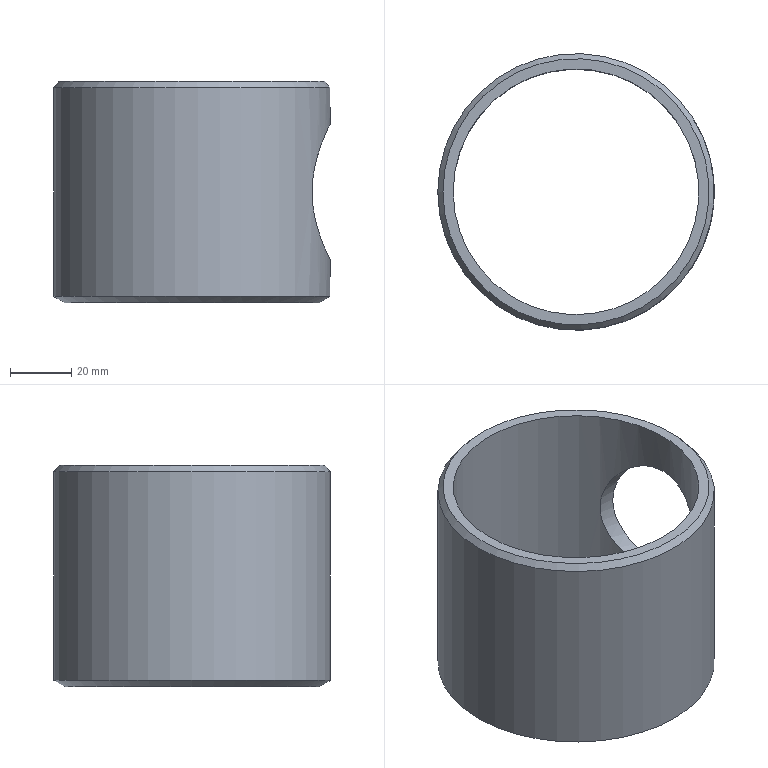Component | NX | CH3404_19_3-3 | 1 solid | 7 faces | box 90 x 90 x 72 mm | volume 86640 mm3 | cylinder 3 | cone 2 | plane 2 | commonest cylinder face diameters 90 x1 80 x1 44.5 x1
STEP:
#1=CARTESIAN_POINT('',(0.,0.,0.));
#2=DIRECTION('',(0.,0.,1.));
#3=DIRECTION('',(1.,0.,0.));
#4=AXIS2_PLACEMENT_3D('',#1,#2,#3);
#5=CARTESIAN_POINT('',(-45.,0.,74.));
#6=VERTEX_POINT('',#5);
#7=CARTESIAN_POINT('',(0.,0.,74.));
#8=DIRECTION('',(0.,0.,-1.));
#9=DIRECTION('',(-1.,0.,0.));
#10=AXIS2_PLACEMENT_3D('',#7,#8,#9);
#11=CIRCLE('',#10,45.);
#12=CARTESIAN_POINT('',(0.,0.,4.));
#13=DIRECTION('',(0.,0.,-1.));
#14=DIRECTION('',(-1.,0.,0.));
#15=AXIS2_PLACEMENT_3D('',#12,#13,#14);
#16=CYLINDRICAL_SURFACE('',#15,45.);
#17=CARTESIAN_POINT('',(0.,-70.));
#18=DIRECTION('',(1.,0.));
#19=VECTOR('',#18,1.);
#20=LINE('',#17,#19);
#21=(GEOMETRIC_REPRESENTATION_CONTEXT(2)PARAMETRIC_REPRESENTATION_CONTEXT()REPRESENTATION_CONTEXT('',''));
#22=DEFINITIONAL_REPRESENTATION('',(#20),#21);
#23=PCURVE('',#16,#22);
#24=CARTESIAN_POINT('',(0.,0.,76.));
#25=DIRECTION('',(0.,0.,-1.));
#26=DIRECTION('',(-1.,0.,0.));
#27=AXIS2_PLACEMENT_3D('',#24,#25,#26);
#28=CONICAL_SURFACE('',#27,43.322,0.6981);
#29=CARTESIAN_POINT('',(0.,2.));
#30=DIRECTION('',(1.,0.));
#31=VECTOR('',#30,1.);
#32=LINE('',#29,#31);
#33=(GEOMETRIC_REPRESENTATION_CONTEXT(2)PARAMETRIC_REPRESENTATION_CONTEXT()REPRESENTATION_CONTEXT('',''));
#34=DEFINITIONAL_REPRESENTATION('',(#32),#33);
#35=PCURVE('',#28,#34);
#36=SURFACE_CURVE('',#11,(#23,#35),.PCURVE_S1.);
#37=EDGE_CURVE('',#6,#6,#36,.T.);
#38=ORIENTED_EDGE('',*,*,#37,.T.);
#39=CARTESIAN_POINT('',(-45.,0.,6.));
#40=VERTEX_POINT('',#39);
#41=CARTESIAN_POINT('',(-45.,0.,74.));
#42=CARTESIAN_POINT('',(-45.,0.,6.));
#43=B_SPLINE_CURVE_WITH_KNOTS('',1,(#41,#42),.UNSPECIFIED.,.F.,.F.,(2,2),(-70.,-2.),.PIECEWISE_BEZIER_KNOTS.);
#44=CARTESIAN_POINT('',(6.283,0.));
#45=DIRECTION('',(0.,1.));
#46=VECTOR('',#45,1.);
#47=LINE('',#44,#46);
#48=(GEOMETRIC_REPRESENTATION_CONTEXT(2)PARAMETRIC_REPRESENTATION_CONTEXT()REPRESENTATION_CONTEXT('',''));
#49=DEFINITIONAL_REPRESENTATION('',(#47),#48);
#50=PCURVE('',#16,#49);
#51=CARTESIAN_POINT('',(0.,0.));
#52=DIRECTION('',(0.,1.));
#53=VECTOR('',#52,1.);
#54=LINE('',#51,#53);
#55=(GEOMETRIC_REPRESENTATION_CONTEXT(2)PARAMETRIC_REPRESENTATION_CONTEXT()REPRESENTATION_CONTEXT('',''));
#56=DEFINITIONAL_REPRESENTATION('',(#54),#55);
#57=PCURVE('',#16,#56);
#58=SEAM_CURVE('',#43,(#50,#57),.PCURVE_S1.);
#59=EDGE_CURVE('',#6,#40,#58,.T.);
#60=ORIENTED_EDGE('',*,*,#59,.T.);
#61=CARTESIAN_POINT('',(0.,0.,6.));
#62=DIRECTION('',(0.,0.,-1.));
#63=DIRECTION('',(-1.,0.,0.));
#64=AXIS2_PLACEMENT_3D('',#61,#62,#63);
#65=CIRCLE('',#64,45.);
#66=CARTESIAN_POINT('',(0.,-2.));
#67=DIRECTION('',(1.,0.));
#68=VECTOR('',#67,1.);
#69=LINE('',#66,#68);
#70=(GEOMETRIC_REPRESENTATION_CONTEXT(2)PARAMETRIC_REPRESENTATION_CONTEXT()REPRESENTATION_CONTEXT('',''));
#71=DEFINITIONAL_REPRESENTATION('',(#69),#70);
#72=PCURVE('',#16,#71);
#73=CARTESIAN_POINT('',(0.,0.,6.));
#74=DIRECTION('',(0.,0.,1.));
#75=DIRECTION('',(1.,0.,0.));
#76=AXIS2_PLACEMENT_3D('',#73,#74,#75);
#77=CONICAL_SURFACE('',#76,45.,1.047);
#78=CARTESIAN_POINT('',(9.425,0.));
#79=DIRECTION('',(-1.,0.));
#80=VECTOR('',#79,1.);
#81=LINE('',#78,#80);
#82=(GEOMETRIC_REPRESENTATION_CONTEXT(2)PARAMETRIC_REPRESENTATION_CONTEXT()REPRESENTATION_CONTEXT('',''));
#83=DEFINITIONAL_REPRESENTATION('',(#81),#82);
#84=PCURVE('',#77,#83);
#85=SURFACE_CURVE('',#65,(#72,#84),.PCURVE_S1.);
#86=EDGE_CURVE('',#40,#40,#85,.T.);
#87=ORIENTED_EDGE('',*,*,#86,.F.);
#88=ORIENTED_EDGE('',*,*,#59,.F.);
#89=EDGE_LOOP('',(#38,#60,#87,#88));
#90=FACE_BOUND('',#89,.T.);
#91=CARTESIAN_POINT('',(45.,0.,62.25));
#92=VERTEX_POINT('',#91);
#93=CARTESIAN_POINT('',(45.,2.991,62.25));
#94=CARTESIAN_POINT('',(45.,-2.991,62.25));
#95=CARTESIAN_POINT('',(44.693,-5.921,61.644));
#96=CARTESIAN_POINT('',(43.646,-11.292,59.392));
#97=CARTESIAN_POINT('',(42.91,-13.724,57.744));
#98=CARTESIAN_POINT('',(41.405,-17.756,53.708));
#99=CARTESIAN_POINT('',(40.626,-19.394,51.281));
#100=CARTESIAN_POINT('',(39.48,-21.631,45.957));
#101=CARTESIAN_POINT('',(39.118,-22.243,43.008));
#102=CARTESIAN_POINT('',(39.111,-22.257,37.093));
#103=CARTESIAN_POINT('',(39.464,-21.66,34.132));
#104=CARTESIAN_POINT('',(40.617,-19.412,28.742));
#105=CARTESIAN_POINT('',(41.395,-17.778,26.32));
#106=CARTESIAN_POINT('',(42.902,-13.75,22.276));
#107=CARTESIAN_POINT('',(43.64,-11.311,20.622));
#108=CARTESIAN_POINT('',(44.684,-5.978,18.374));
#109=CARTESIAN_POINT('',(44.996,-3.009,17.758));
#110=CARTESIAN_POINT('',(45.004,2.891,17.742));
#111=CARTESIAN_POINT('',(44.704,5.848,18.332));
#112=CARTESIAN_POINT('',(43.652,11.275,20.594));
#113=CARTESIAN_POINT('',(42.919,13.697,22.233));
#114=CARTESIAN_POINT('',(41.408,17.751,26.282));
#115=CARTESIAN_POINT('',(40.628,19.39,28.711));
#116=CARTESIAN_POINT('',(39.481,21.629,34.035));
#117=CARTESIAN_POINT('',(39.118,22.243,37.003));
#118=CARTESIAN_POINT('',(39.111,22.257,42.892));
#119=CARTESIAN_POINT('',(39.464,21.661,45.861));
#120=CARTESIAN_POINT('',(40.614,19.418,51.247));
#121=CARTESIAN_POINT('',(41.392,17.788,53.672));
#122=CARTESIAN_POINT('',(42.911,13.725,57.747));
#123=CARTESIAN_POINT('',(43.643,11.303,59.385));
#124=CARTESIAN_POINT('',(44.69,5.936,61.64));
#125=CARTESIAN_POINT('',(45.,2.991,62.25));
#126=CARTESIAN_POINT('',(45.,-2.991,62.25));
#127=B_SPLINE_CURVE_WITH_KNOTS('',3,(#93,#94,#95,#96,#97,#98,#99,#100,#101,#102,#103,#104,#105,#106,#107,#108,#109,#110,#111,#112,#113,#114,#115,#116,#117,#118,#119,#120,#121,#122,#123,#124,#125,#126),.UNSPECIFIED.,.T.,.F.,(2,2,2,2,2,2,2,2,2,2,2,2,2,2,2,2,2,2,2),(-0.0625,0.,0.0625,0.125,0.1875,0.25,0.3125,0.375,0.4375,0.5,0.5625,0.625,0.6875,0.75,0.8125,0.875,0.9375,1.,1.062),.UNSPECIFIED.);
#128=CARTESIAN_POINT('',(3.142,-58.25));
#129=CARTESIAN_POINT('',(3.158,-58.25));
#130=CARTESIAN_POINT('',(3.19,-58.179));
#131=CARTESIAN_POINT('',(3.237,-57.866));
#132=CARTESIAN_POINT('',(3.284,-57.354));
#133=CARTESIAN_POINT('',(3.329,-56.65));
#134=CARTESIAN_POINT('',(3.372,-55.761));
#135=CARTESIAN_POINT('',(3.414,-54.7));
#136=CARTESIAN_POINT('',(3.454,-53.479));
#137=CARTESIAN_POINT('',(3.491,-52.111));
#138=CARTESIAN_POINT('',(3.525,-50.608));
#139=CARTESIAN_POINT('',(3.556,-48.97));
#140=CARTESIAN_POINT('',(3.584,-47.214));
#141=CARTESIAN_POINT('',(3.608,-45.354));
#142=CARTESIAN_POINT('',(3.627,-43.405));
#143=CARTESIAN_POINT('',(3.643,-41.367));
#144=CARTESIAN_POINT('',(3.653,-39.266));
#145=CARTESIAN_POINT('',(3.659,-37.127));
#146=CARTESIAN_POINT('',(3.659,-34.974));
#147=CARTESIAN_POINT('',(3.654,-32.83));
#148=CARTESIAN_POINT('',(3.643,-30.72));
#149=CARTESIAN_POINT('',(3.628,-28.666));
#150=CARTESIAN_POINT('',(3.608,-26.692));
#151=CARTESIAN_POINT('',(3.584,-24.819));
#152=CARTESIAN_POINT('',(3.556,-23.057));
#153=CARTESIAN_POINT('',(3.525,-21.417));
#154=CARTESIAN_POINT('',(3.491,-19.912));
#155=CARTESIAN_POINT('',(3.454,-18.541));
#156=CARTESIAN_POINT('',(3.415,-17.317));
#157=CARTESIAN_POINT('',(3.373,-16.254));
#158=CARTESIAN_POINT('',(3.33,-15.367));
#159=CARTESIAN_POINT('',(3.285,-14.662));
#160=CARTESIAN_POINT('',(3.238,-14.146));
#161=CARTESIAN_POINT('',(3.191,-13.827));
#162=CARTESIAN_POINT('',(3.143,-13.715));
#163=CARTESIAN_POINT('',(3.095,-13.815));
#164=CARTESIAN_POINT('',(3.048,-14.12));
#165=CARTESIAN_POINT('',(3.001,-14.627));
#166=CARTESIAN_POINT('',(2.955,-15.331));
#167=CARTESIAN_POINT('',(2.911,-16.222));
#168=CARTESIAN_POINT('',(2.87,-17.282));
#169=CARTESIAN_POINT('',(2.83,-18.502));
#170=CARTESIAN_POINT('',(2.793,-19.871));
#171=CARTESIAN_POINT('',(2.759,-21.379));
#172=CARTESIAN_POINT('',(2.727,-23.02));
#173=CARTESIAN_POINT('',(2.7,-24.778));
#174=CARTESIAN_POINT('',(2.676,-26.638));
#175=CARTESIAN_POINT('',(2.656,-28.587));
#176=CARTESIAN_POINT('',(2.64,-30.631));
#177=CARTESIAN_POINT('',(2.63,-32.736));
#178=CARTESIAN_POINT('',(2.624,-34.876));
#179=CARTESIAN_POINT('',(2.624,-37.02));
#180=CARTESIAN_POINT('',(2.629,-39.16));
#181=CARTESIAN_POINT('',(2.64,-41.271));
#182=CARTESIAN_POINT('',(2.655,-43.326));
#183=CARTESIAN_POINT('',(2.675,-45.299));
#184=CARTESIAN_POINT('',(2.699,-47.171));
#185=CARTESIAN_POINT('',(2.727,-48.936));
#186=CARTESIAN_POINT('',(2.758,-50.581));
#187=CARTESIAN_POINT('',(2.792,-52.099));
#188=CARTESIAN_POINT('',(2.829,-53.474));
#189=CARTESIAN_POINT('',(2.869,-54.696));
#190=CARTESIAN_POINT('',(2.911,-55.756));
#191=CARTESIAN_POINT('',(2.954,-56.644));
#192=CARTESIAN_POINT('',(2.999,-57.35));
#193=CARTESIAN_POINT('',(3.046,-57.864));
#194=CARTESIAN_POINT('',(3.093,-58.178));
#195=CARTESIAN_POINT('',(3.125,-58.25));
#196=CARTESIAN_POINT('',(3.142,-58.25));
#197=B_SPLINE_CURVE_WITH_KNOTS('',3,(#128,#129,#130,#131,#132,#133,#134,#135,#136,#137,#138,#139,#140,#141,#142,#143,#144,#145,#146,#147,#148,#149,#150,#151,#152,#153,#154,#155,#156,#157,#158,#159,#160,#161,#162,#163,#164,#165,#166,#167,#168,#169,#170,#171,#172,#173,#174,#175,#176,#177,#178,#179,#180,#181,#182,#183,#184,#185,#186,#187,#188,#189,#190,#191,#192,#193,#194,#195,#196),.UNSPECIFIED.,.T.,.F.,(4,1,1,1,1,1,1,1,1,1,1,1,1,1,1,1,1,1,1,1,1,1,1,1,1,1,1,1,1,1,1,1,1,1,1,1,1,1,1,1,1,1,1,1,1,1,1,1,1,1,1,1,1,1,1,1,1,1,1,1,1,1,1,1,1,1,4),(0.,0.01515,0.0303,0.04545,0.06061,0.07576,0.09091,0.1061,0.1212,0.1364,0.1515,0.1667,0.1818,0.197,0.2121,0.2273,0.2424,0.2576,0.2727,0.2879,0.303,0.3182,0.3333,0.3485,0.3636,0.3788,0.3939,0.4091,0.4242,0.4394,0.4545,0.4697,0.4848,0.5,0.5152,0.5303,0.5455,0.5606,0.5758,0.5909,0.6061,0.6212,0.6364,0.6515,0.6667,0.6818,0.697,0.7121,0.7273,0.7424,0.7576,0.7727,0.7879,0.803,0.8182,0.8333,0.8485,0.8636,0.8788,0.8939,0.9091,0.9242,0.9394,0.9545,0.9697,0.9848,1.),.QUASI_UNIFORM_KNOTS.);
#198=(GEOMETRIC_REPRESENTATION_CONTEXT(2)PARAMETRIC_REPRESENTATION_CONTEXT()REPRESENTATION_CONTEXT('',''));
#199=DEFINITIONAL_REPRESENTATION('',(#197),#198);
#200=PCURVE('',#16,#199);
#201=CARTESIAN_POINT('',(49.5,0.,40.));
#202=DIRECTION('',(-1.,0.,0.));
#203=DIRECTION('',(0.,0.,1.));
#204=AXIS2_PLACEMENT_3D('',#201,#202,#203);
#205=CYLINDRICAL_SURFACE('',#204,22.25);
#206=CARTESIAN_POINT('',(6.283,4.5));
#207=CARTESIAN_POINT('',(6.251,4.5));
#208=CARTESIAN_POINT('',(6.186,4.536));
#209=CARTESIAN_POINT('',(6.089,4.691));
#210=CARTESIAN_POINT('',(5.993,4.938));
#211=CARTESIAN_POINT('',(5.898,5.271));
#212=CARTESIAN_POINT('',(5.803,5.68));
#213=CARTESIAN_POINT('',(5.708,6.15));
#214=CARTESIAN_POINT('',(5.614,6.664));
#215=CARTESIAN_POINT('',(5.521,7.204));
#216=CARTESIAN_POINT('',(5.427,7.755));
#217=CARTESIAN_POINT('',(5.334,8.301));
#218=CARTESIAN_POINT('',(5.24,8.822));
#219=CARTESIAN_POINT('',(5.146,9.297));
#220=CARTESIAN_POINT('',(5.051,9.706));
#221=CARTESIAN_POINT('',(4.956,10.033));
#222=CARTESIAN_POINT('',(4.86,10.264));
#223=CARTESIAN_POINT('',(4.763,10.389));
#224=CARTESIAN_POINT('',(4.666,10.392));
#225=CARTESIAN_POINT('',(4.57,10.272));
#226=CARTESIAN_POINT('',(4.473,10.045));
#227=CARTESIAN_POINT('',(4.377,9.72));
#228=CARTESIAN_POINT('',(4.281,9.308));
#229=CARTESIAN_POINT('',(4.187,8.831));
#230=CARTESIAN_POINT('',(4.093,8.311));
#231=CARTESIAN_POINT('',(3.999,7.764));
#232=CARTESIAN_POINT('',(3.906,7.213));
#233=CARTESIAN_POINT('',(3.812,6.672));
#234=CARTESIAN_POINT('',(3.718,6.158));
#235=CARTESIAN_POINT('',(3.623,5.687));
#236=CARTESIAN_POINT('',(3.529,5.279));
#237=CARTESIAN_POINT('',(3.434,4.946));
#238=CARTESIAN_POINT('',(3.337,4.697));
#239=CARTESIAN_POINT('',(3.241,4.539));
#240=CARTESIAN_POINT('',(3.144,4.482));
#241=CARTESIAN_POINT('',(3.048,4.533));
#242=CARTESIAN_POINT('',(2.951,4.684));
#243=CARTESIAN_POINT('',(2.855,4.929));
#244=CARTESIAN_POINT('',(2.759,5.262));
#245=CARTESIAN_POINT('',(2.663,5.673));
#246=CARTESIAN_POINT('',(2.568,6.143));
#247=CARTESIAN_POINT('',(2.474,6.656));
#248=CARTESIAN_POINT('',(2.38,7.197));
#249=CARTESIAN_POINT('',(2.287,7.751));
#250=CARTESIAN_POINT('',(2.193,8.298));
#251=CARTESIAN_POINT('',(2.099,8.819));
#252=CARTESIAN_POINT('',(2.004,9.295));
#253=CARTESIAN_POINT('',(1.91,9.705));
#254=CARTESIAN_POINT('',(1.814,10.032));
#255=CARTESIAN_POINT('',(1.718,10.264));
#256=CARTESIAN_POINT('',(1.621,10.389));
#257=CARTESIAN_POINT('',(1.525,10.392));
#258=CARTESIAN_POINT('',(1.428,10.273));
#259=CARTESIAN_POINT('',(1.332,10.045));
#260=CARTESIAN_POINT('',(1.236,9.721));
#261=CARTESIAN_POINT('',(1.14,9.31));
#262=CARTESIAN_POINT('',(1.046,8.834));
#263=CARTESIAN_POINT('',(0.9514,8.313));
#264=CARTESIAN_POINT('',(0.8574,7.765));
#265=CARTESIAN_POINT('',(0.7634,7.209));
#266=CARTESIAN_POINT('',(0.6694,6.666));
#267=CARTESIAN_POINT('',(0.5753,6.152));
#268=CARTESIAN_POINT('',(0.4809,5.683));
#269=CARTESIAN_POINT('',(0.386,5.273));
#270=CARTESIAN_POINT('',(0.2905,4.94));
#271=CARTESIAN_POINT('',(0.1943,4.692));
#272=CARTESIAN_POINT('',(0.09753,4.536));
#273=CARTESIAN_POINT('',(0.03258,4.5));
#274=CARTESIAN_POINT('',(0.,4.5));
#275=B_SPLINE_CURVE_WITH_KNOTS('',3,(#206,#207,#208,#209,#210,#211,#212,#213,#214,#215,#216,#217,#218,#219,#220,#221,#222,#223,#224,#225,#226,#227,#228,#229,#230,#231,#232,#233,#234,#235,#236,#237,#238,#239,#240,#241,#242,#243,#244,#245,#246,#247,#248,#249,#250,#251,#252,#253,#254,#255,#256,#257,#258,#259,#260,#261,#262,#263,#264,#265,#266,#267,#268,#269,#270,#271,#272,#273,#274),.UNSPECIFIED.,.F.,.F.,(4,1,1,1,1,1,1,1,1,1,1,1,1,1,1,1,1,1,1,1,1,1,1,1,1,1,1,1,1,1,1,1,1,1,1,1,1,1,1,1,1,1,1,1,1,1,1,1,1,1,1,1,1,1,1,1,1,1,1,1,1,1,1,1,1,1,4),(0.,0.01515,0.0303,0.04545,0.06061,0.07576,0.09091,0.1061,0.1212,0.1364,0.1515,0.1667,0.1818,0.197,0.2121,0.2273,0.2424,0.2576,0.2727,0.2879,0.303,0.3182,0.3333,0.3485,0.3636,0.3788,0.3939,0.4091,0.4242,0.4394,0.4545,0.4697,0.4848,0.5,0.5152,0.5303,0.5455,0.5606,0.5758,0.5909,0.6061,0.6212,0.6364,0.6515,0.6667,0.6818,0.697,0.7121,0.7273,0.7424,0.7576,0.7727,0.7879,0.803,0.8182,0.8333,0.8485,0.8636,0.8788,0.8939,0.9091,0.9242,0.9394,0.9545,0.9697,0.9848,1.),.QUASI_UNIFORM_KNOTS.);
#276=(GEOMETRIC_REPRESENTATION_CONTEXT(2)PARAMETRIC_REPRESENTATION_CONTEXT()REPRESENTATION_CONTEXT('',''));
#277=DEFINITIONAL_REPRESENTATION('',(#275),#276);
#278=PCURVE('',#205,#277);
#279=SURFACE_CURVE('',#127,(#200,#278),.PCURVE_S1.);
#280=EDGE_CURVE('',#92,#92,#279,.T.);
#281=ORIENTED_EDGE('',*,*,#280,.F.);
#282=EDGE_LOOP('',(#281));
#283=FACE_BOUND('',#282,.T.);
#284=ADVANCED_FACE('',(#90,#283),#16,.T.);
#285=CARTESIAN_POINT('',(-40.,0.,4.));
#286=VERTEX_POINT('',#285);
#287=CARTESIAN_POINT('',(0.,0.,4.));
#288=DIRECTION('',(0.,0.,-1.));
#289=DIRECTION('',(-1.,0.,0.));
#290=AXIS2_PLACEMENT_3D('',#287,#288,#289);
#291=CIRCLE('',#290,40.);
#292=CARTESIAN_POINT('',(0.,0.,4.));
#293=DIRECTION('',(0.,0.,-1.));
#294=DIRECTION('',(-1.,0.,0.));
#295=AXIS2_PLACEMENT_3D('',#292,#293,#294);
#296=CYLINDRICAL_SURFACE('',#295,40.);
#297=CARTESIAN_POINT('',(0.,0.));
#298=DIRECTION('',(1.,0.));
#299=VECTOR('',#298,1.);
#300=LINE('',#297,#299);
#301=(GEOMETRIC_REPRESENTATION_CONTEXT(2)PARAMETRIC_REPRESENTATION_CONTEXT()REPRESENTATION_CONTEXT('',''));
#302=DEFINITIONAL_REPRESENTATION('',(#300),#301);
#303=PCURVE('',#296,#302);
#304=CARTESIAN_POINT('',(0.,-41.536,4.));
#305=DIRECTION('',(0.,0.,1.));
#306=DIRECTION('',(1.,0.,0.));
#307=AXIS2_PLACEMENT_3D('',#304,#305,#306);
#308=PLANE('',#307);
#309=CARTESIAN_POINT('',(-40.,41.536));
#310=CARTESIAN_POINT('',(-40.,110.818));
#311=CARTESIAN_POINT('',(20.,76.177));
#312=CARTESIAN_POINT('',(80.,41.536));
#313=CARTESIAN_POINT('',(20.,6.895));
#314=CARTESIAN_POINT('',(-40.,-27.746));
#315=CARTESIAN_POINT('',(-40.,41.536));
#316=(BOUNDED_CURVE()B_SPLINE_CURVE(2,(#309,#310,#311,#312,#313,#314,#315),.UNSPECIFIED.,.T.,.F.)B_SPLINE_CURVE_WITH_KNOTS((1,2,2,2,2,1),(-2.094,0.,2.094,4.189,6.283,8.378),.UNSPECIFIED.)CURVE()GEOMETRIC_REPRESENTATION_ITEM()RATIONAL_B_SPLINE_CURVE((1.,0.5,1.,0.5,1.,0.5,1.))REPRESENTATION_ITEM(''));
#317=(GEOMETRIC_REPRESENTATION_CONTEXT(2)PARAMETRIC_REPRESENTATION_CONTEXT()REPRESENTATION_CONTEXT('',''));
#318=DEFINITIONAL_REPRESENTATION('',(#316),#317);
#319=PCURVE('',#308,#318);
#320=SURFACE_CURVE('',#291,(#303,#319),.PCURVE_S1.);
#321=EDGE_CURVE('',#286,#286,#320,.T.);
#322=ORIENTED_EDGE('',*,*,#321,.F.);
#323=CARTESIAN_POINT('',(-40.,0.,76.));
#324=VERTEX_POINT('',#323);
#325=CARTESIAN_POINT('',(-40.,-0.,76.));
#326=CARTESIAN_POINT('',(-40.,-0.,4.));
#327=B_SPLINE_CURVE_WITH_KNOTS('',1,(#325,#326),.UNSPECIFIED.,.F.,.F.,(2,2),(-72.,0.),.PIECEWISE_BEZIER_KNOTS.);
#328=CARTESIAN_POINT('',(0.,0.));
#329=DIRECTION('',(0.,1.));
#330=VECTOR('',#329,1.);
#331=LINE('',#328,#330);
#332=(GEOMETRIC_REPRESENTATION_CONTEXT(2)PARAMETRIC_REPRESENTATION_CONTEXT()REPRESENTATION_CONTEXT('',''));
#333=DEFINITIONAL_REPRESENTATION('',(#331),#332);
#334=PCURVE('',#296,#333);
#335=CARTESIAN_POINT('',(6.283,0.));
#336=DIRECTION('',(0.,1.));
#337=VECTOR('',#336,1.);
#338=LINE('',#335,#337);
#339=(GEOMETRIC_REPRESENTATION_CONTEXT(2)PARAMETRIC_REPRESENTATION_CONTEXT()REPRESENTATION_CONTEXT('',''));
#340=DEFINITIONAL_REPRESENTATION('',(#338),#339);
#341=PCURVE('',#296,#340);
#342=SEAM_CURVE('',#327,(#334,#341),.PCURVE_S1.);
#343=EDGE_CURVE('',#324,#286,#342,.T.);
#344=ORIENTED_EDGE('',*,*,#343,.F.);
#345=CARTESIAN_POINT('',(0.,0.,76.));
#346=DIRECTION('',(0.,0.,-1.));
#347=DIRECTION('',(-1.,0.,0.));
#348=AXIS2_PLACEMENT_3D('',#345,#346,#347);
#349=CIRCLE('',#348,40.);
#350=CARTESIAN_POINT('',(0.,-72.));
#351=DIRECTION('',(1.,0.));
#352=VECTOR('',#351,1.);
#353=LINE('',#350,#352);
#354=(GEOMETRIC_REPRESENTATION_CONTEXT(2)PARAMETRIC_REPRESENTATION_CONTEXT()REPRESENTATION_CONTEXT('',''));
#355=DEFINITIONAL_REPRESENTATION('',(#353),#354);
#356=PCURVE('',#296,#355);
#357=CARTESIAN_POINT('',(0.,-40.,76.));
#358=DIRECTION('',(0.,0.,-1.));
#359=DIRECTION('',(-1.,0.,0.));
#360=AXIS2_PLACEMENT_3D('',#357,#358,#359);
#361=PLANE('',#360);
#362=CARTESIAN_POINT('',(0.,40.));
#363=DIRECTION('',(1.,0.));
#364=AXIS2_PLACEMENT_2D('',#362,#363);
#365=CIRCLE('',#364,40.);
#366=(GEOMETRIC_REPRESENTATION_CONTEXT(2)PARAMETRIC_REPRESENTATION_CONTEXT()REPRESENTATION_CONTEXT('',''));
#367=DEFINITIONAL_REPRESENTATION('',(#365),#366);
#368=PCURVE('',#361,#367);
#369=SURFACE_CURVE('',#349,(#356,#368),.PCURVE_S1.);
#370=EDGE_CURVE('',#324,#324,#369,.T.);
#371=ORIENTED_EDGE('',*,*,#370,.T.);
#372=ORIENTED_EDGE('',*,*,#343,.T.);
#373=EDGE_LOOP('',(#322,#344,#371,#372));
#374=FACE_BOUND('',#373,.F.);
#375=CARTESIAN_POINT('',(40.,-0.,62.25));
#376=VERTEX_POINT('',#375);
#377=CARTESIAN_POINT('',(40.,-3.006,62.25));
#378=CARTESIAN_POINT('',(40.,3.006,62.25));
#379=CARTESIAN_POINT('',(39.65,5.95,61.637));
#380=CARTESIAN_POINT('',(38.464,11.318,59.377));
#381=CARTESIAN_POINT('',(37.63,13.739,57.73));
#382=CARTESIAN_POINT('',(35.912,17.751,53.712));
#383=CARTESIAN_POINT('',(35.017,19.379,51.306));
#384=CARTESIAN_POINT('',(33.679,21.621,45.993));
#385=CARTESIAN_POINT('',(33.244,22.245,43.043));
#386=CARTESIAN_POINT('',(33.237,22.255,37.028));
#387=CARTESIAN_POINT('',(33.664,21.643,34.08));
#388=CARTESIAN_POINT('',(35.002,19.404,28.733));
#389=CARTESIAN_POINT('',(35.899,17.778,26.321));
#390=CARTESIAN_POINT('',(37.62,13.765,22.289));
#391=CARTESIAN_POINT('',(38.451,11.359,20.648));
#392=CARTESIAN_POINT('',(39.643,5.997,18.376));
#393=CARTESIAN_POINT('',(39.996,3.059,17.758));
#394=CARTESIAN_POINT('',(40.004,-2.942,17.742));
#395=CARTESIAN_POINT('',(39.657,-5.907,18.351));
#396=CARTESIAN_POINT('',(38.472,-11.291,20.607));
#397=CARTESIAN_POINT('',(37.638,-13.718,22.253));
#398=CARTESIAN_POINT('',(35.918,-17.74,26.272));
#399=CARTESIAN_POINT('',(35.021,-19.371,28.679));
#400=CARTESIAN_POINT('',(33.679,-21.62,34.001));
#401=CARTESIAN_POINT('',(33.244,-22.246,36.957));
#402=CARTESIAN_POINT('',(33.238,-22.254,42.979));
#403=CARTESIAN_POINT('',(33.666,-21.641,45.93));
#404=CARTESIAN_POINT('',(35.007,-19.396,51.281));
#405=CARTESIAN_POINT('',(35.905,-17.766,53.695));
#406=CARTESIAN_POINT('',(37.63,-13.741,57.731));
#407=CARTESIAN_POINT('',(38.46,-11.333,59.369));
#408=CARTESIAN_POINT('',(39.651,-5.952,61.637));
#409=CARTESIAN_POINT('',(40.,-3.006,62.25));
#410=CARTESIAN_POINT('',(40.,3.006,62.25));
#411=B_SPLINE_CURVE_WITH_KNOTS('',3,(#377,#378,#379,#380,#381,#382,#383,#384,#385,#386,#387,#388,#389,#390,#391,#392,#393,#394,#395,#396,#397,#398,#399,#400,#401,#402,#403,#404,#405,#406,#407,#408,#409,#410),.UNSPECIFIED.,.T.,.F.,(2,2,2,2,2,2,2,2,2,2,2,2,2,2,2,2,2,2,2),(-0.0625,0.,0.0625,0.125,0.1875,0.25,0.3125,0.375,0.4375,0.5,0.5625,0.625,0.6875,0.75,0.8125,0.875,0.9375,1.,1.062),.UNSPECIFIED.);
#412=CARTESIAN_POINT('',(3.142,-58.25));
#413=CARTESIAN_POINT('',(3.123,-58.25));
#414=CARTESIAN_POINT('',(3.087,-58.178));
#415=CARTESIAN_POINT('',(3.034,-57.862));
#416=CARTESIAN_POINT('',(2.981,-57.346));
#417=CARTESIAN_POINT('',(2.93,-56.639));
#418=CARTESIAN_POINT('',(2.881,-55.748));
#419=CARTESIAN_POINT('',(2.833,-54.686));
#420=CARTESIAN_POINT('',(2.789,-53.467));
#421=CARTESIAN_POINT('',(2.747,-52.105));
#422=CARTESIAN_POINT('',(2.708,-50.609));
#423=CARTESIAN_POINT('',(2.672,-48.981));
#424=CARTESIAN_POINT('',(2.64,-47.235));
#425=CARTESIAN_POINT('',(2.612,-45.384));
#426=CARTESIAN_POINT('',(2.589,-43.438));
#427=CARTESIAN_POINT('',(2.571,-41.4));
#428=CARTESIAN_POINT('',(2.558,-39.29));
#429=CARTESIAN_POINT('',(2.552,-37.132));
#430=CARTESIAN_POINT('',(2.551,-34.939));
#431=CARTESIAN_POINT('',(2.558,-32.78));
#432=CARTESIAN_POINT('',(2.57,-30.67));
#433=CARTESIAN_POINT('',(2.588,-28.626));
#434=CARTESIAN_POINT('',(2.611,-26.668));
#435=CARTESIAN_POINT('',(2.639,-24.807));
#436=CARTESIAN_POINT('',(2.671,-23.055));
#437=CARTESIAN_POINT('',(2.707,-21.421));
#438=CARTESIAN_POINT('',(2.746,-19.92));
#439=CARTESIAN_POINT('',(2.788,-18.555));
#440=CARTESIAN_POINT('',(2.833,-17.335));
#441=CARTESIAN_POINT('',(2.88,-16.274));
#442=CARTESIAN_POINT('',(2.929,-15.38));
#443=CARTESIAN_POINT('',(2.98,-14.668));
#444=CARTESIAN_POINT('',(3.032,-14.148));
#445=CARTESIAN_POINT('',(3.086,-13.828));
#446=CARTESIAN_POINT('',(3.14,-13.714));
#447=CARTESIAN_POINT('',(3.195,-13.817));
#448=CARTESIAN_POINT('',(3.248,-14.129));
#449=CARTESIAN_POINT('',(3.301,-14.642));
#450=CARTESIAN_POINT('',(3.352,-15.347));
#451=CARTESIAN_POINT('',(3.402,-16.236));
#452=CARTESIAN_POINT('',(3.449,-17.297));
#453=CARTESIAN_POINT('',(3.494,-18.516));
#454=CARTESIAN_POINT('',(3.536,-19.879));
#455=CARTESIAN_POINT('',(3.575,-21.375));
#456=CARTESIAN_POINT('',(3.611,-23.004));
#457=CARTESIAN_POINT('',(3.643,-24.751));
#458=CARTESIAN_POINT('',(3.671,-26.605));
#459=CARTESIAN_POINT('',(3.694,-28.553));
#460=CARTESIAN_POINT('',(3.712,-30.596));
#461=CARTESIAN_POINT('',(3.725,-32.708));
#462=CARTESIAN_POINT('',(3.732,-34.87));
#463=CARTESIAN_POINT('',(3.732,-37.066));
#464=CARTESIAN_POINT('',(3.725,-39.227));
#465=CARTESIAN_POINT('',(3.713,-41.34));
#466=CARTESIAN_POINT('',(3.695,-43.386));
#467=CARTESIAN_POINT('',(3.672,-45.345));
#468=CARTESIAN_POINT('',(3.644,-47.207));
#469=CARTESIAN_POINT('',(3.612,-48.961));
#470=CARTESIAN_POINT('',(3.576,-50.596));
#471=CARTESIAN_POINT('',(3.537,-52.098));
#472=CARTESIAN_POINT('',(3.495,-53.464));
#473=CARTESIAN_POINT('',(3.45,-54.682));
#474=CARTESIAN_POINT('',(3.403,-55.742));
#475=CARTESIAN_POINT('',(3.353,-56.635));
#476=CARTESIAN_POINT('',(3.302,-57.345));
#477=CARTESIAN_POINT('',(3.25,-57.862));
#478=CARTESIAN_POINT('',(3.196,-58.178));
#479=CARTESIAN_POINT('',(3.16,-58.25));
#480=CARTESIAN_POINT('',(3.142,-58.25));
#481=B_SPLINE_CURVE_WITH_KNOTS('',3,(#412,#413,#414,#415,#416,#417,#418,#419,#420,#421,#422,#423,#424,#425,#426,#427,#428,#429,#430,#431,#432,#433,#434,#435,#436,#437,#438,#439,#440,#441,#442,#443,#444,#445,#446,#447,#448,#449,#450,#451,#452,#453,#454,#455,#456,#457,#458,#459,#460,#461,#462,#463,#464,#465,#466,#467,#468,#469,#470,#471,#472,#473,#474,#475,#476,#477,#478,#479,#480),.UNSPECIFIED.,.T.,.F.,(4,1,1,1,1,1,1,1,1,1,1,1,1,1,1,1,1,1,1,1,1,1,1,1,1,1,1,1,1,1,1,1,1,1,1,1,1,1,1,1,1,1,1,1,1,1,1,1,1,1,1,1,1,1,1,1,1,1,1,1,1,1,1,1,1,1,4),(0.,0.01515,0.0303,0.04545,0.06061,0.07576,0.09091,0.1061,0.1212,0.1364,0.1515,0.1667,0.1818,0.197,0.2121,0.2273,0.2424,0.2576,0.2727,0.2879,0.303,0.3182,0.3333,0.3485,0.3636,0.3788,0.3939,0.4091,0.4242,0.4394,0.4545,0.4697,0.4848,0.5,0.5152,0.5303,0.5455,0.5606,0.5758,0.5909,0.6061,0.6212,0.6364,0.6515,0.6667,0.6818,0.697,0.7121,0.7273,0.7424,0.7576,0.7727,0.7879,0.803,0.8182,0.8333,0.8485,0.8636,0.8788,0.8939,0.9091,0.9242,0.9394,0.9545,0.9697,0.9848,1.),.QUASI_UNIFORM_KNOTS.);
#482=(GEOMETRIC_REPRESENTATION_CONTEXT(2)PARAMETRIC_REPRESENTATION_CONTEXT()REPRESENTATION_CONTEXT('',''));
#483=DEFINITIONAL_REPRESENTATION('',(#481),#482);
#484=PCURVE('',#296,#483);
#485=CARTESIAN_POINT('',(0.,9.5));
#486=CARTESIAN_POINT('',(0.03275,9.5));
#487=CARTESIAN_POINT('',(0.09794,9.541));
#488=CARTESIAN_POINT('',(0.1949,9.717));
#489=CARTESIAN_POINT('',(0.2911,9.998));
#490=CARTESIAN_POINT('',(0.3867,10.375));
#491=CARTESIAN_POINT('',(0.4816,10.839));
#492=CARTESIAN_POINT('',(0.576,11.372));
#493=CARTESIAN_POINT('',(0.6698,11.956));
#494=CARTESIAN_POINT('',(0.763,12.571));
#495=CARTESIAN_POINT('',(0.8557,13.2));
#496=CARTESIAN_POINT('',(0.9489,13.826));
#497=CARTESIAN_POINT('',(1.042,14.426));
#498=CARTESIAN_POINT('',(1.136,14.977));
#499=CARTESIAN_POINT('',(1.23,15.455));
#500=CARTESIAN_POINT('',(1.326,15.84));
#501=CARTESIAN_POINT('',(1.423,16.115));
#502=CARTESIAN_POINT('',(1.52,16.264));
#503=CARTESIAN_POINT('',(1.618,16.266));
#504=CARTESIAN_POINT('',(1.716,16.122));
#505=CARTESIAN_POINT('',(1.812,15.852));
#506=CARTESIAN_POINT('',(1.908,15.47));
#507=CARTESIAN_POINT('',(2.003,14.991));
#508=CARTESIAN_POINT('',(2.097,14.44));
#509=CARTESIAN_POINT('',(2.191,13.84));
#510=CARTESIAN_POINT('',(2.284,13.212));
#511=CARTESIAN_POINT('',(2.377,12.582));
#512=CARTESIAN_POINT('',(2.47,11.966));
#513=CARTESIAN_POINT('',(2.564,11.383));
#514=CARTESIAN_POINT('',(2.658,10.85));
#515=CARTESIAN_POINT('',(2.753,10.385));
#516=CARTESIAN_POINT('',(2.848,10.006));
#517=CARTESIAN_POINT('',(2.944,9.722));
#518=CARTESIAN_POINT('',(3.041,9.544));
#519=CARTESIAN_POINT('',(3.139,9.479));
#520=CARTESIAN_POINT('',(3.237,9.538));
#521=CARTESIAN_POINT('',(3.334,9.712));
#522=CARTESIAN_POINT('',(3.431,9.991));
#523=CARTESIAN_POINT('',(3.527,10.367));
#524=CARTESIAN_POINT('',(3.622,10.831));
#525=CARTESIAN_POINT('',(3.716,11.364));
#526=CARTESIAN_POINT('',(3.81,11.948));
#527=CARTESIAN_POINT('',(3.904,12.564));
#528=CARTESIAN_POINT('',(3.996,13.194));
#529=CARTESIAN_POINT('',(4.09,13.821));
#530=CARTESIAN_POINT('',(4.183,14.422));
#531=CARTESIAN_POINT('',(4.277,14.973));
#532=CARTESIAN_POINT('',(4.372,15.454));
#533=CARTESIAN_POINT('',(4.467,15.84));
#534=CARTESIAN_POINT('',(4.564,16.115));
#535=CARTESIAN_POINT('',(4.662,16.264));
#536=CARTESIAN_POINT('',(4.76,16.266));
#537=CARTESIAN_POINT('',(4.858,16.122));
#538=CARTESIAN_POINT('',(4.954,15.85));
#539=CARTESIAN_POINT('',(5.05,15.467));
#540=CARTESIAN_POINT('',(5.145,14.987));
#541=CARTESIAN_POINT('',(5.239,14.435));
#542=CARTESIAN_POINT('',(5.333,13.834));
#543=CARTESIAN_POINT('',(5.427,13.206));
#544=CARTESIAN_POINT('',(5.52,12.574));
#545=CARTESIAN_POINT('',(5.613,11.958));
#546=CARTESIAN_POINT('',(5.707,11.375));
#547=CARTESIAN_POINT('',(5.801,10.842));
#548=CARTESIAN_POINT('',(5.896,10.377));
#549=CARTESIAN_POINT('',(5.992,9.999));
#550=CARTESIAN_POINT('',(6.088,9.717));
#551=CARTESIAN_POINT('',(6.185,9.541));
#552=CARTESIAN_POINT('',(6.25,9.5));
#553=CARTESIAN_POINT('',(6.283,9.5));
#554=B_SPLINE_CURVE_WITH_KNOTS('',3,(#485,#486,#487,#488,#489,#490,#491,#492,#493,#494,#495,#496,#497,#498,#499,#500,#501,#502,#503,#504,#505,#506,#507,#508,#509,#510,#511,#512,#513,#514,#515,#516,#517,#518,#519,#520,#521,#522,#523,#524,#525,#526,#527,#528,#529,#530,#531,#532,#533,#534,#535,#536,#537,#538,#539,#540,#541,#542,#543,#544,#545,#546,#547,#548,#549,#550,#551,#552,#553),.UNSPECIFIED.,.F.,.F.,(4,1,1,1,1,1,1,1,1,1,1,1,1,1,1,1,1,1,1,1,1,1,1,1,1,1,1,1,1,1,1,1,1,1,1,1,1,1,1,1,1,1,1,1,1,1,1,1,1,1,1,1,1,1,1,1,1,1,1,1,1,1,1,1,1,1,4),(0.,0.01515,0.0303,0.04545,0.06061,0.07576,0.09091,0.1061,0.1212,0.1364,0.1515,0.1667,0.1818,0.197,0.2121,0.2273,0.2424,0.2576,0.2727,0.2879,0.303,0.3182,0.3333,0.3485,0.3636,0.3788,0.3939,0.4091,0.4242,0.4394,0.4545,0.4697,0.4848,0.5,0.5152,0.5303,0.5455,0.5606,0.5758,0.5909,0.6061,0.6212,0.6364,0.6515,0.6667,0.6818,0.697,0.7121,0.7273,0.7424,0.7576,0.7727,0.7879,0.803,0.8182,0.8333,0.8485,0.8636,0.8788,0.8939,0.9091,0.9242,0.9394,0.9545,0.9697,0.9848,1.),.QUASI_UNIFORM_KNOTS.);
#555=(GEOMETRIC_REPRESENTATION_CONTEXT(2)PARAMETRIC_REPRESENTATION_CONTEXT()REPRESENTATION_CONTEXT('',''));
#556=DEFINITIONAL_REPRESENTATION('',(#554),#555);
#557=PCURVE('',#205,#556);
#558=SURFACE_CURVE('',#411,(#484,#557),.PCURVE_S1.);
#559=EDGE_CURVE('',#376,#376,#558,.T.);
#560=ORIENTED_EDGE('',*,*,#559,.T.);
#561=EDGE_LOOP('',(#560));
#562=FACE_BOUND('',#561,.F.);
#563=ADVANCED_FACE('',(#374,#562),#296,.F.);
#564=CARTESIAN_POINT('',(-41.536,0.,4.));
#565=VERTEX_POINT('',#564);
#566=CARTESIAN_POINT('',(0.,0.,4.));
#567=DIRECTION('',(0.,0.,-1.));
#568=DIRECTION('',(-1.,0.,0.));
#569=AXIS2_PLACEMENT_3D('',#566,#567,#568);
#570=CIRCLE('',#569,41.536);
#571=CARTESIAN_POINT('',(9.425,-2.));
#572=DIRECTION('',(-1.,0.));
#573=VECTOR('',#572,1.);
#574=LINE('',#571,#573);
#575=(GEOMETRIC_REPRESENTATION_CONTEXT(2)PARAMETRIC_REPRESENTATION_CONTEXT()REPRESENTATION_CONTEXT('',''));
#576=DEFINITIONAL_REPRESENTATION('',(#574),#575);
#577=PCURVE('',#77,#576);
#578=CARTESIAN_POINT('',(-41.536,41.536));
#579=CARTESIAN_POINT('',(-41.536,113.478));
#580=CARTESIAN_POINT('',(20.768,77.507));
#581=CARTESIAN_POINT('',(83.072,41.536));
#582=CARTESIAN_POINT('',(20.768,5.565));
#583=CARTESIAN_POINT('',(-41.536,-30.406));
#584=CARTESIAN_POINT('',(-41.536,41.536));
#585=(BOUNDED_CURVE()B_SPLINE_CURVE(2,(#578,#579,#580,#581,#582,#583,#584),.UNSPECIFIED.,.T.,.F.)B_SPLINE_CURVE_WITH_KNOTS((1,2,2,2,2,1),(-2.094,0.,2.094,4.189,6.283,8.378),.UNSPECIFIED.)CURVE()GEOMETRIC_REPRESENTATION_ITEM()RATIONAL_B_SPLINE_CURVE((1.,0.5,1.,0.5,1.,0.5,1.))REPRESENTATION_ITEM(''));
#586=(GEOMETRIC_REPRESENTATION_CONTEXT(2)PARAMETRIC_REPRESENTATION_CONTEXT()REPRESENTATION_CONTEXT('',''));
#587=DEFINITIONAL_REPRESENTATION('',(#585),#586);
#588=PCURVE('',#308,#587);
#589=SURFACE_CURVE('',#570,(#577,#588),.PCURVE_S1.);
#590=EDGE_CURVE('',#565,#565,#589,.T.);
#591=ORIENTED_EDGE('',*,*,#590,.F.);
#592=CARTESIAN_POINT('',(-41.536,0.,4.));
#593=CARTESIAN_POINT('',(-45.,0.,6.));
#594=B_SPLINE_CURVE_WITH_KNOTS('',1,(#592,#593),.UNSPECIFIED.,.F.,.F.,(2,2),(-4.,0.),.PIECEWISE_BEZIER_KNOTS.);
#595=CARTESIAN_POINT('',(9.425,0.));
#596=DIRECTION('',(0.,1.));
#597=VECTOR('',#596,1.);
#598=LINE('',#595,#597);
#599=(GEOMETRIC_REPRESENTATION_CONTEXT(2)PARAMETRIC_REPRESENTATION_CONTEXT()REPRESENTATION_CONTEXT('',''));
#600=DEFINITIONAL_REPRESENTATION('',(#598),#599);
#601=PCURVE('',#77,#600);
#602=CARTESIAN_POINT('',(3.142,0.));
#603=DIRECTION('',(0.,1.));
#604=VECTOR('',#603,1.);
#605=LINE('',#602,#604);
#606=(GEOMETRIC_REPRESENTATION_CONTEXT(2)PARAMETRIC_REPRESENTATION_CONTEXT()REPRESENTATION_CONTEXT('',''));
#607=DEFINITIONAL_REPRESENTATION('',(#605),#606);
#608=PCURVE('',#77,#607);
#609=SEAM_CURVE('',#594,(#601,#608),.PCURVE_S1.);
#610=EDGE_CURVE('',#565,#40,#609,.T.);
#611=ORIENTED_EDGE('',*,*,#610,.T.);
#612=ORIENTED_EDGE('',*,*,#86,.T.);
#613=ORIENTED_EDGE('',*,*,#610,.F.);
#614=EDGE_LOOP('',(#591,#611,#612,#613));
#615=FACE_BOUND('',#614,.T.);
#616=ADVANCED_FACE('',(#615),#77,.T.);
#617=ORIENTED_EDGE('',*,*,#321,.F.);
#618=EDGE_LOOP('',(#617));
#619=FACE_BOUND('',#618,.T.);
#620=ORIENTED_EDGE('',*,*,#590,.T.);
#621=EDGE_LOOP('',(#620));
#622=FACE_BOUND('',#621,.T.);
#623=ADVANCED_FACE('',(#619,#622),#308,.F.);
#624=CARTESIAN_POINT('',(-43.322,0.,76.));
#625=VERTEX_POINT('',#624);
#626=CARTESIAN_POINT('',(0.,0.,76.));
#627=DIRECTION('',(0.,0.,-1.));
#628=DIRECTION('',(-1.,0.,0.));
#629=AXIS2_PLACEMENT_3D('',#626,#627,#628);
#630=CIRCLE('',#629,43.322);
#631=CARTESIAN_POINT('',(0.,40.));
#632=DIRECTION('',(1.,0.));
#633=AXIS2_PLACEMENT_2D('',#631,#632);
#634=CIRCLE('',#633,43.322);
#635=(GEOMETRIC_REPRESENTATION_CONTEXT(2)PARAMETRIC_REPRESENTATION_CONTEXT()REPRESENTATION_CONTEXT('',''));
#636=DEFINITIONAL_REPRESENTATION('',(#634),#635);
#637=PCURVE('',#361,#636);
#638=CARTESIAN_POINT('',(0.,0.));
#639=DIRECTION('',(1.,0.));
#640=VECTOR('',#639,1.);
#641=LINE('',#638,#640);
#642=(GEOMETRIC_REPRESENTATION_CONTEXT(2)PARAMETRIC_REPRESENTATION_CONTEXT()REPRESENTATION_CONTEXT('',''));
#643=DEFINITIONAL_REPRESENTATION('',(#641),#642);
#644=PCURVE('',#28,#643);
#645=SURFACE_CURVE('',#630,(#637,#644),.PCURVE_S1.);
#646=EDGE_CURVE('',#625,#625,#645,.T.);
#647=ORIENTED_EDGE('',*,*,#646,.F.);
#648=EDGE_LOOP('',(#647));
#649=FACE_BOUND('',#648,.T.);
#650=ORIENTED_EDGE('',*,*,#370,.T.);
#651=EDGE_LOOP('',(#650));
#652=FACE_BOUND('',#651,.T.);
#653=ADVANCED_FACE('',(#649,#652),#361,.F.);
#654=ORIENTED_EDGE('',*,*,#37,.F.);
#655=CARTESIAN_POINT('',(-43.322,-0.,76.));
#656=CARTESIAN_POINT('',(-45.,-0.,74.));
#657=B_SPLINE_CURVE_WITH_KNOTS('',1,(#655,#656),.UNSPECIFIED.,.F.,.F.,(2,2),(0.,2.611),.PIECEWISE_BEZIER_KNOTS.);
#658=CARTESIAN_POINT('',(0.,0.));
#659=DIRECTION('',(0.,1.));
#660=VECTOR('',#659,1.);
#661=LINE('',#658,#660);
#662=(GEOMETRIC_REPRESENTATION_CONTEXT(2)PARAMETRIC_REPRESENTATION_CONTEXT()REPRESENTATION_CONTEXT('',''));
#663=DEFINITIONAL_REPRESENTATION('',(#661),#662);
#664=PCURVE('',#28,#663);
#665=CARTESIAN_POINT('',(6.283,0.));
#666=DIRECTION('',(0.,1.));
#667=VECTOR('',#666,1.);
#668=LINE('',#665,#667);
#669=(GEOMETRIC_REPRESENTATION_CONTEXT(2)PARAMETRIC_REPRESENTATION_CONTEXT()REPRESENTATION_CONTEXT('',''));
#670=DEFINITIONAL_REPRESENTATION('',(#668),#669);
#671=PCURVE('',#28,#670);
#672=SEAM_CURVE('',#657,(#664,#671),.PCURVE_S1.);
#673=EDGE_CURVE('',#625,#6,#672,.T.);
#674=ORIENTED_EDGE('',*,*,#673,.F.);
#675=ORIENTED_EDGE('',*,*,#646,.T.);
#676=ORIENTED_EDGE('',*,*,#673,.T.);
#677=EDGE_LOOP('',(#654,#674,#675,#676));
#678=FACE_BOUND('',#677,.T.);
#679=ADVANCED_FACE('',(#678),#28,.T.);
#680=ORIENTED_EDGE('',*,*,#559,.F.);
#681=CARTESIAN_POINT('',(45.,-0.,62.25));
#682=CARTESIAN_POINT('',(40.,-0.,62.25));
#683=B_SPLINE_CURVE_WITH_KNOTS('',1,(#681,#682),.UNSPECIFIED.,.F.,.F.,(2,2),(4.5,9.5),.PIECEWISE_BEZIER_KNOTS.);
#684=CARTESIAN_POINT('',(0.,0.));
#685=DIRECTION('',(0.,1.));
#686=VECTOR('',#685,1.);
#687=LINE('',#684,#686);
#688=(GEOMETRIC_REPRESENTATION_CONTEXT(2)PARAMETRIC_REPRESENTATION_CONTEXT()REPRESENTATION_CONTEXT('',''));
#689=DEFINITIONAL_REPRESENTATION('',(#687),#688);
#690=PCURVE('',#205,#689);
#691=CARTESIAN_POINT('',(6.283,0.));
#692=DIRECTION('',(0.,1.));
#693=VECTOR('',#692,1.);
#694=LINE('',#691,#693);
#695=(GEOMETRIC_REPRESENTATION_CONTEXT(2)PARAMETRIC_REPRESENTATION_CONTEXT()REPRESENTATION_CONTEXT('',''));
#696=DEFINITIONAL_REPRESENTATION('',(#694),#695);
#697=PCURVE('',#205,#696);
#698=SEAM_CURVE('',#683,(#690,#697),.PCURVE_S1.);
#699=EDGE_CURVE('',#92,#376,#698,.T.);
#700=ORIENTED_EDGE('',*,*,#699,.F.);
#701=ORIENTED_EDGE('',*,*,#280,.F.);
#702=ORIENTED_EDGE('',*,*,#699,.T.);
#703=EDGE_LOOP('',(#680,#700,#701,#702));
#704=FACE_BOUND('',#703,.F.);
#705=ADVANCED_FACE('',(#704),#205,.F.);
#706=CLOSED_SHELL('',(#284,#563,#616,#623,#653,#679,#705));
#707=MANIFOLD_SOLID_BREP('',#706);
#708=(LENGTH_UNIT()NAMED_UNIT(*)SI_UNIT(.MILLI.,.METRE.));
#709=UNCERTAINTY_MEASURE_WITH_UNIT(LENGTH_MEASURE(0.0005),#708,'','');
#710=(NAMED_UNIT(*)PLANE_ANGLE_UNIT()SI_UNIT($,.RADIAN.));
#711=(NAMED_UNIT(*)SI_UNIT($,.STERADIAN.)SOLID_ANGLE_UNIT());
#712=(GEOMETRIC_REPRESENTATION_CONTEXT(3)GLOBAL_UNCERTAINTY_ASSIGNED_CONTEXT((#709))GLOBAL_UNIT_ASSIGNED_CONTEXT((#708,#710,#711))REPRESENTATION_CONTEXT('',''));
#713=ADVANCED_BREP_SHAPE_REPRESENTATION('',(#4,#707),#712);